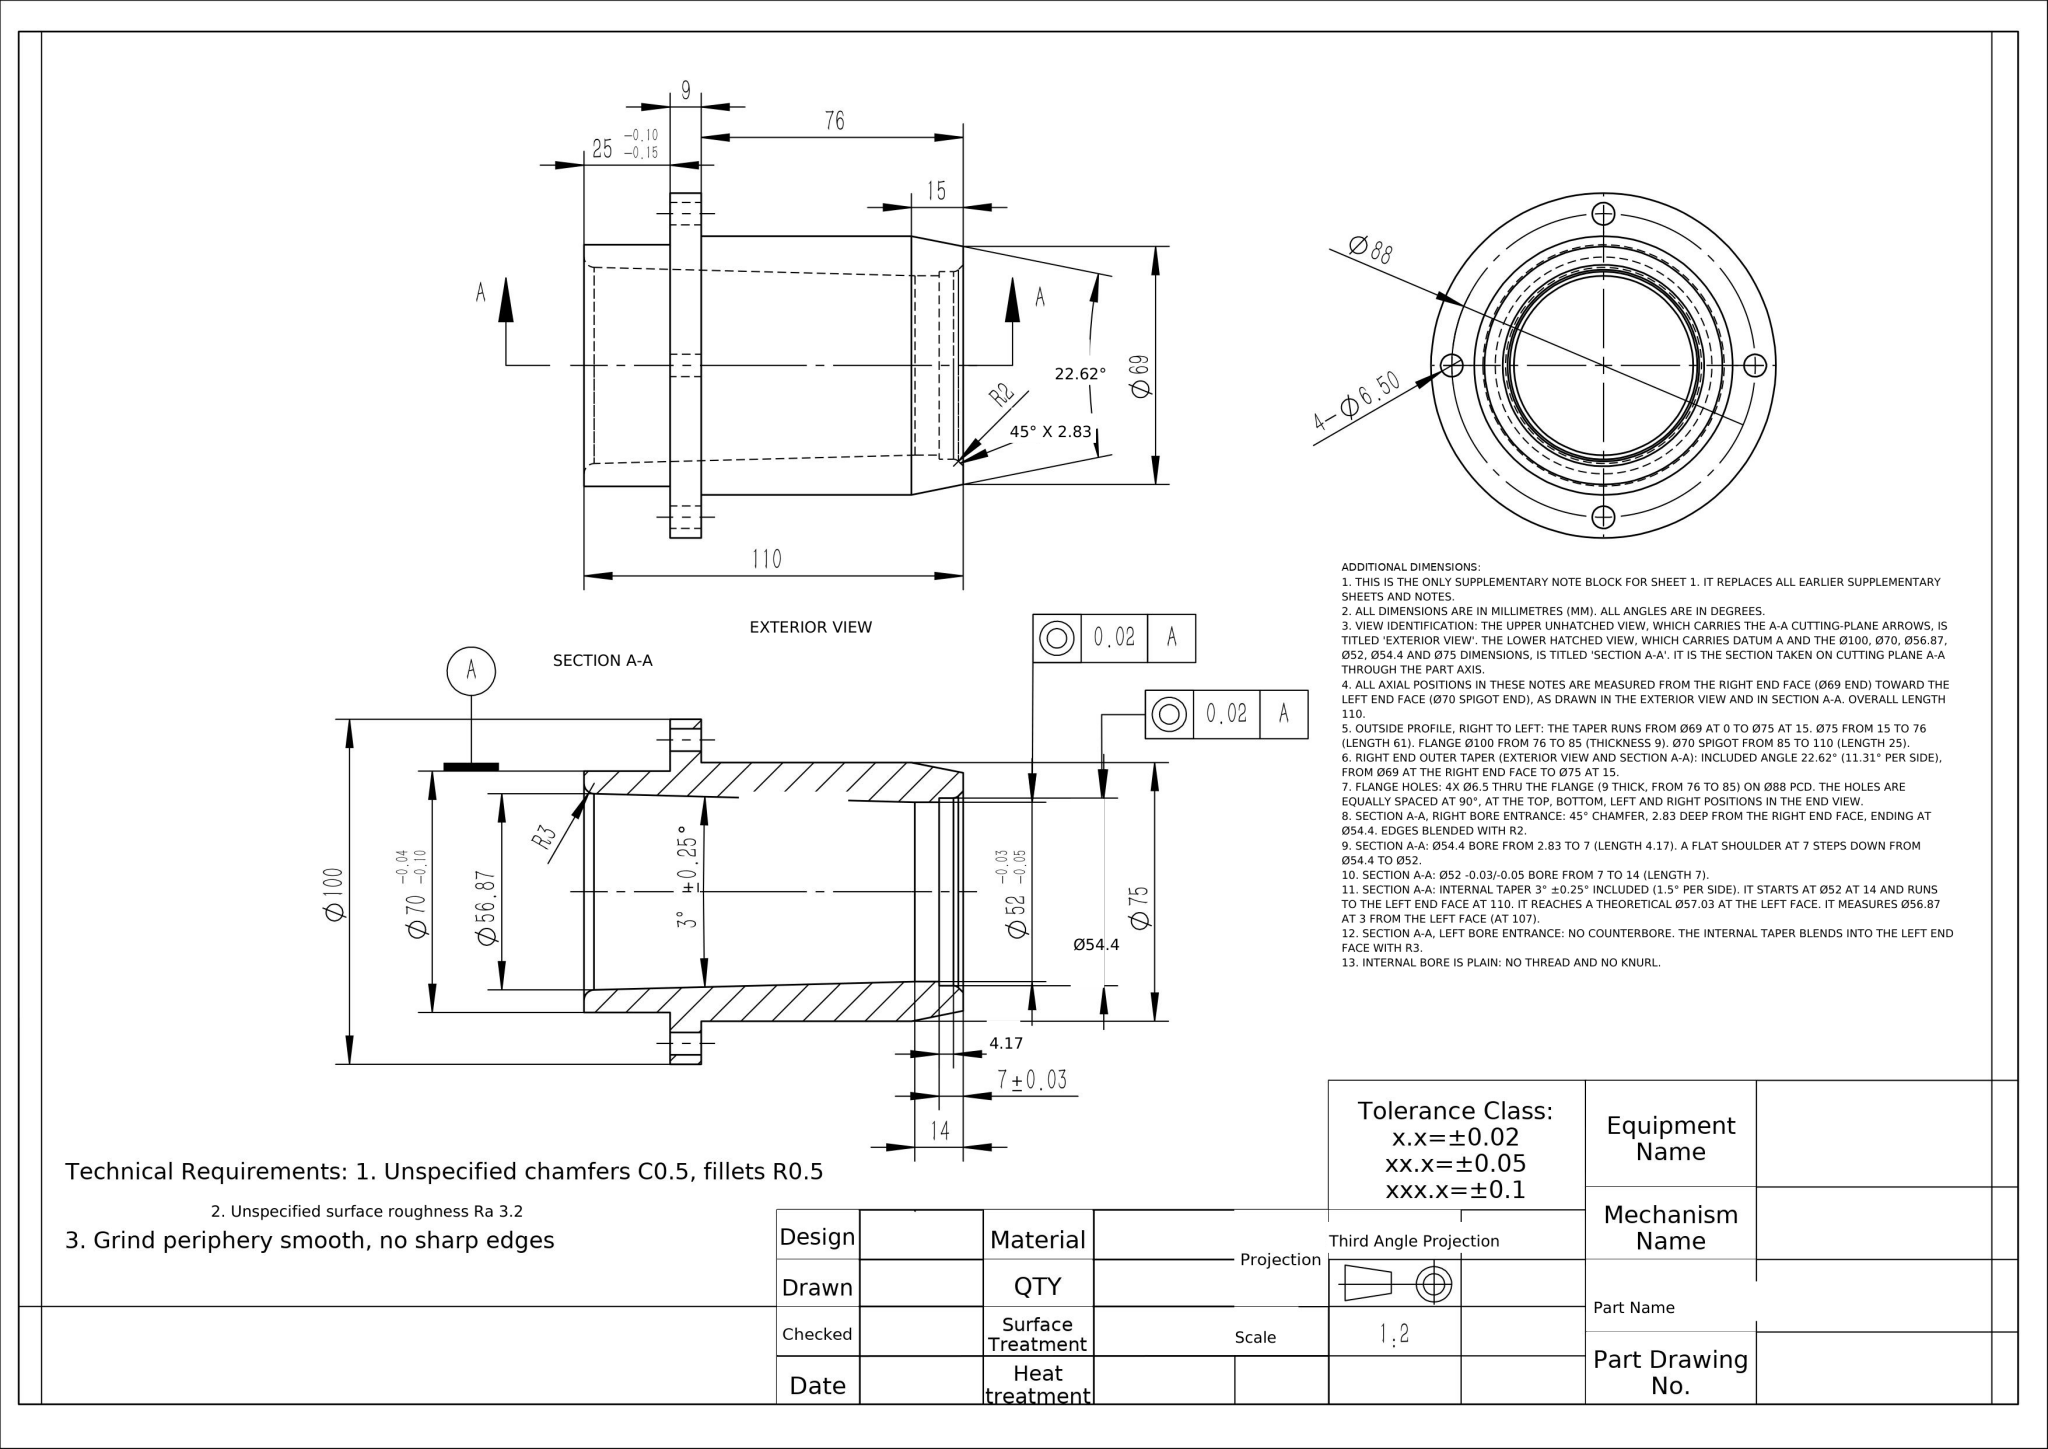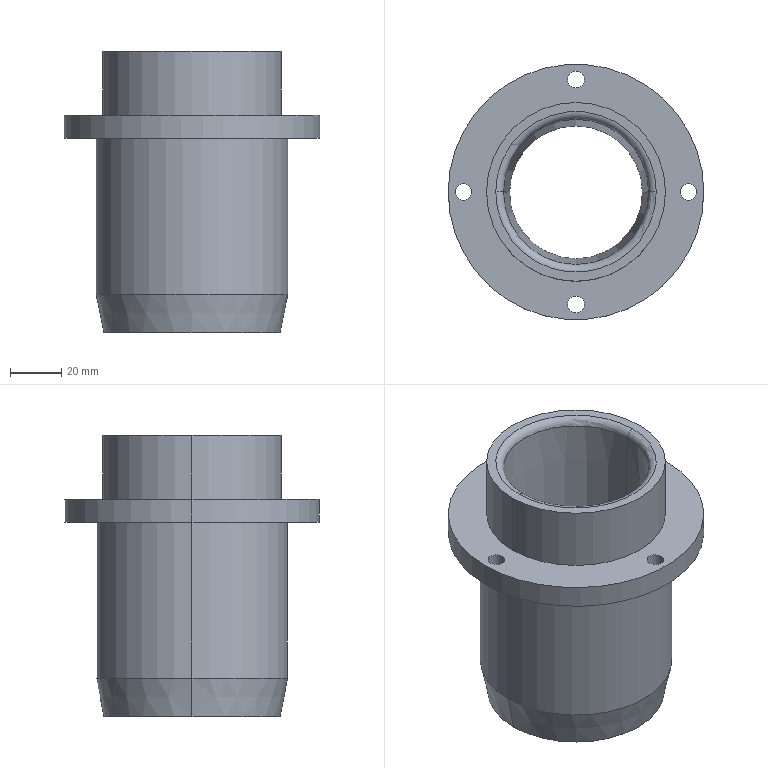Part | NX | mm | 1 solid | 33 faces | box 100 x 100 x 110 mm | volume 240242 mm3 | cylinder 18 | cone 6 | plane 5 | torus 4 | commonest cylinder face diameters 6.5 x8 54.4 x2 70 x2 100 x2 75 x2 52 x2
STEP:
#1=CARTESIAN_POINT('',(-27.2,0.,2.828));
#2=VERTEX_POINT('',#1);
#3=CARTESIAN_POINT('',(27.2,0.,2.828));
#4=VERTEX_POINT('',#3);
#5=CARTESIAN_POINT('',(0.,0.,2.828));
#6=DIRECTION('',(0.,0.,-1.));
#7=DIRECTION('',(1.,0.,0.));
#8=AXIS2_PLACEMENT_3D('',#5,#6,#7);
#9=CIRCLE('',#8,27.2);
#10=EDGE_CURVE('',#2,#4,#9,.T.);
#11=ORIENTED_EDGE('',*,*,#10,.F.);
#12=CARTESIAN_POINT('',(-27.786,0.,1.414));
#13=VERTEX_POINT('',#12);
#14=CARTESIAN_POINT('',(-29.2,0.,2.828));
#15=DIRECTION('',(0.,1.,0.));
#16=DIRECTION('',(-1.,0.,0.));
#17=AXIS2_PLACEMENT_3D('',#14,#15,#16);
#18=CIRCLE('',#17,2.);
#19=EDGE_CURVE('',#2,#13,#18,.T.);
#20=ORIENTED_EDGE('',*,*,#19,.T.);
#21=CARTESIAN_POINT('',(27.786,0.,1.414));
#22=VERTEX_POINT('',#21);
#23=CARTESIAN_POINT('',(0.,0.,1.414));
#24=DIRECTION('',(0.,0.,1.));
#25=DIRECTION('',(-1.,0.,0.));
#26=AXIS2_PLACEMENT_3D('',#23,#24,#25);
#27=CIRCLE('',#26,27.786);
#28=EDGE_CURVE('',#22,#13,#27,.T.);
#29=ORIENTED_EDGE('',*,*,#28,.F.);
#30=CARTESIAN_POINT('',(29.2,0.,2.828));
#31=DIRECTION('',(0.,-1.,0.));
#32=DIRECTION('',(0.,0.,-1.));
#33=AXIS2_PLACEMENT_3D('',#30,#31,#32);
#34=CIRCLE('',#33,2.);
#35=EDGE_CURVE('',#4,#22,#34,.T.);
#36=ORIENTED_EDGE('',*,*,#35,.F.);
#37=EDGE_LOOP('',(#11,#20,#29,#36));
#38=FACE_OUTER_BOUND('',#37,.T.);
#39=CARTESIAN_POINT('',(0.,0.,2.828));
#40=DIRECTION('',(0.,0.,1.));
#41=DIRECTION('',(1.,0.,0.));
#42=AXIS2_PLACEMENT_3D('',#39,#40,#41);
#43=TOROIDAL_SURFACE('',#42,29.2,2.);
#44=ADVANCED_FACE('',(#38),#43,.T.);
#45=CARTESIAN_POINT('',(-34.5,0.,0.));
#46=VERTEX_POINT('',#45);
#47=CARTESIAN_POINT('',(34.5,0.,0.));
#48=VERTEX_POINT('',#47);
#49=CARTESIAN_POINT('',(0.,0.,0.));
#50=DIRECTION('',(0.,0.,-1.));
#51=DIRECTION('',(1.,0.,0.));
#52=AXIS2_PLACEMENT_3D('',#49,#50,#51);
#53=CIRCLE('',#52,34.5);
#54=EDGE_CURVE('',#46,#48,#53,.T.);
#55=ORIENTED_EDGE('',*,*,#54,.F.);
#56=CARTESIAN_POINT('',(-37.5,0.,15.));
#57=VERTEX_POINT('',#56);
#58=CARTESIAN_POINT('',(-37.5,0.,15.));
#59=DIRECTION('',(-0.1961,0.,0.9806));
#60=VECTOR('',#59,1000.);
#61=LINE('',#58,#60);
#62=EDGE_CURVE('',#46,#57,#61,.T.);
#63=ORIENTED_EDGE('',*,*,#62,.T.);
#64=CARTESIAN_POINT('',(37.5,0.,15.));
#65=VERTEX_POINT('',#64);
#66=CARTESIAN_POINT('',(0.,0.,15.));
#67=DIRECTION('',(0.,0.,1.));
#68=DIRECTION('',(1.,0.,0.));
#69=AXIS2_PLACEMENT_3D('',#66,#67,#68);
#70=CIRCLE('',#69,37.5);
#71=EDGE_CURVE('',#65,#57,#70,.T.);
#72=ORIENTED_EDGE('',*,*,#71,.F.);
#73=CARTESIAN_POINT('',(37.5,0.,15.));
#74=DIRECTION('',(0.1961,0.,0.9806));
#75=VECTOR('',#74,1000.);
#76=LINE('',#73,#75);
#77=EDGE_CURVE('',#48,#65,#76,.T.);
#78=ORIENTED_EDGE('',*,*,#77,.F.);
#79=EDGE_LOOP('',(#55,#63,#72,#78));
#80=FACE_OUTER_BOUND('',#79,.T.);
#81=CARTESIAN_POINT('',(0.,0.,15.));
#82=DIRECTION('',(0.,0.,1.));
#83=DIRECTION('',(1.,0.,0.));
#84=AXIS2_PLACEMENT_3D('',#81,#82,#83);
#85=CONICAL_SURFACE('',#84,37.5,0.1974);
#86=ADVANCED_FACE('',(#80),#85,.T.);
#87=CARTESIAN_POINT('',(0.,0.,1.414));
#88=DIRECTION('',(0.,0.,1.));
#89=DIRECTION('',(-1.,0.,0.));
#90=AXIS2_PLACEMENT_3D('',#87,#88,#89);
#91=CIRCLE('',#90,27.786);
#92=EDGE_CURVE('',#13,#22,#91,.T.);
#93=ORIENTED_EDGE('',*,*,#92,.T.);
#94=CARTESIAN_POINT('',(29.2,0.,0.));
#95=VERTEX_POINT('',#94);
#96=CARTESIAN_POINT('',(27.2,0.,2.));
#97=DIRECTION('',(0.7071,0.,-0.7071));
#98=VECTOR('',#97,1000.);
#99=LINE('',#96,#98);
#100=EDGE_CURVE('',#22,#95,#99,.T.);
#101=ORIENTED_EDGE('',*,*,#100,.T.);
#102=CARTESIAN_POINT('',(-29.2,0.,0.));
#103=VERTEX_POINT('',#102);
#104=CARTESIAN_POINT('',(0.,0.,0.));
#105=DIRECTION('',(0.,0.,1.));
#106=DIRECTION('',(1.,0.,0.));
#107=AXIS2_PLACEMENT_3D('',#104,#105,#106);
#108=CIRCLE('',#107,29.2);
#109=EDGE_CURVE('',#103,#95,#108,.T.);
#110=ORIENTED_EDGE('',*,*,#109,.F.);
#111=CARTESIAN_POINT('',(-27.2,0.,2.));
#112=DIRECTION('',(-0.7071,0.,-0.7071));
#113=VECTOR('',#112,1000.);
#114=LINE('',#111,#113);
#115=EDGE_CURVE('',#13,#103,#114,.T.);
#116=ORIENTED_EDGE('',*,*,#115,.F.);
#117=EDGE_LOOP('',(#93,#101,#110,#116));
#118=FACE_OUTER_BOUND('',#117,.T.);
#119=CARTESIAN_POINT('',(0.,0.,2.));
#120=DIRECTION('',(0.,0.,-1.));
#121=DIRECTION('',(-1.,0.,0.));
#122=AXIS2_PLACEMENT_3D('',#119,#120,#121);
#123=CONICAL_SURFACE('',#122,27.2,0.7854);
#124=ADVANCED_FACE('',(#118),#123,.F.);
#125=CARTESIAN_POINT('',(-31.436,0.,110.));
#126=VERTEX_POINT('',#125);
#127=CARTESIAN_POINT('',(31.436,0.,110.));
#128=VERTEX_POINT('',#127);
#129=CARTESIAN_POINT('',(0.,0.,110.));
#130=DIRECTION('',(0.,0.,-1.));
#131=DIRECTION('',(1.,0.,0.));
#132=AXIS2_PLACEMENT_3D('',#129,#130,#131);
#133=CIRCLE('',#132,31.436);
#134=EDGE_CURVE('',#126,#128,#133,.T.);
#135=ORIENTED_EDGE('',*,*,#134,.F.);
#136=CARTESIAN_POINT('',(-28.437,0.,107.079));
#137=VERTEX_POINT('',#136);
#138=CARTESIAN_POINT('',(-31.436,0.,107.));
#139=DIRECTION('',(0.,1.,0.));
#140=DIRECTION('',(-1.,0.,0.));
#141=AXIS2_PLACEMENT_3D('',#138,#139,#140);
#142=CIRCLE('',#141,3.);
#143=EDGE_CURVE('',#126,#137,#142,.T.);
#144=ORIENTED_EDGE('',*,*,#143,.T.);
#145=CARTESIAN_POINT('',(28.437,0.,107.079));
#146=VERTEX_POINT('',#145);
#147=CARTESIAN_POINT('',(0.,0.,107.079));
#148=DIRECTION('',(0.,0.,1.));
#149=DIRECTION('',(-1.,0.,0.));
#150=AXIS2_PLACEMENT_3D('',#147,#148,#149);
#151=CIRCLE('',#150,28.437);
#152=EDGE_CURVE('',#146,#137,#151,.T.);
#153=ORIENTED_EDGE('',*,*,#152,.F.);
#154=CARTESIAN_POINT('',(31.436,0.,107.));
#155=DIRECTION('',(0.,-1.,0.));
#156=DIRECTION('',(0.,0.,-1.));
#157=AXIS2_PLACEMENT_3D('',#154,#155,#156);
#158=CIRCLE('',#157,3.);
#159=EDGE_CURVE('',#128,#146,#158,.T.);
#160=ORIENTED_EDGE('',*,*,#159,.F.);
#161=EDGE_LOOP('',(#135,#144,#153,#160));
#162=FACE_OUTER_BOUND('',#161,.T.);
#163=CARTESIAN_POINT('',(0.,0.,107.));
#164=DIRECTION('',(0.,0.,1.));
#165=DIRECTION('',(1.,0.,0.));
#166=AXIS2_PLACEMENT_3D('',#163,#164,#165);
#167=TOROIDAL_SURFACE('',#166,31.436,3.);
#168=ADVANCED_FACE('',(#162),#167,.T.);
#169=CARTESIAN_POINT('',(26.,0.,14.));
#170=VERTEX_POINT('',#169);
#171=CARTESIAN_POINT('',(-26.,0.,14.));
#172=VERTEX_POINT('',#171);
#173=CARTESIAN_POINT('',(0.,0.,14.));
#174=DIRECTION('',(0.,0.,-1.));
#175=DIRECTION('',(-1.,0.,0.));
#176=AXIS2_PLACEMENT_3D('',#173,#174,#175);
#177=CIRCLE('',#176,26.);
#178=EDGE_CURVE('',#170,#172,#177,.T.);
#179=ORIENTED_EDGE('',*,*,#178,.T.);
#180=CARTESIAN_POINT('',(-28.514,0.,110.));
#181=DIRECTION('',(-0.02618,0.,0.9997));
#182=VECTOR('',#181,1000.);
#183=LINE('',#180,#182);
#184=EDGE_CURVE('',#172,#137,#183,.T.);
#185=ORIENTED_EDGE('',*,*,#184,.T.);
#186=CARTESIAN_POINT('',(0.,0.,107.079));
#187=DIRECTION('',(0.,0.,1.));
#188=DIRECTION('',(-1.,0.,0.));
#189=AXIS2_PLACEMENT_3D('',#186,#187,#188);
#190=CIRCLE('',#189,28.437);
#191=EDGE_CURVE('',#137,#146,#190,.T.);
#192=ORIENTED_EDGE('',*,*,#191,.T.);
#193=CARTESIAN_POINT('',(28.514,0.,110.));
#194=DIRECTION('',(0.02618,0.,0.9997));
#195=VECTOR('',#194,1000.);
#196=LINE('',#193,#195);
#197=EDGE_CURVE('',#170,#146,#196,.T.);
#198=ORIENTED_EDGE('',*,*,#197,.F.);
#199=EDGE_LOOP('',(#179,#185,#192,#198));
#200=FACE_OUTER_BOUND('',#199,.T.);
#201=CARTESIAN_POINT('',(0.,0.,110.));
#202=DIRECTION('',(0.,0.,1.));
#203=DIRECTION('',(1.,0.,0.));
#204=AXIS2_PLACEMENT_3D('',#201,#202,#203);
#205=CONICAL_SURFACE('',#204,28.514,0.02618);
#206=ADVANCED_FACE('',(#200),#205,.F.);
#207=CARTESIAN_POINT('',(-3.25,44.,76.));
#208=VERTEX_POINT('',#207);
#209=CARTESIAN_POINT('',(3.25,44.,76.));
#210=VERTEX_POINT('',#209);
#211=CARTESIAN_POINT('',(0.,44.,76.));
#212=DIRECTION('',(0.,0.,1.));
#213=DIRECTION('',(1.,0.,0.));
#214=AXIS2_PLACEMENT_3D('',#211,#212,#213);
#215=CIRCLE('',#214,3.25);
#216=EDGE_CURVE('',#208,#210,#215,.T.);
#217=ORIENTED_EDGE('',*,*,#216,.F.);
#218=CARTESIAN_POINT('',(-3.25,44.,85.));
#219=VERTEX_POINT('',#218);
#220=CARTESIAN_POINT('',(-3.25,44.,85.));
#221=DIRECTION('',(0.,0.,1.));
#222=VECTOR('',#221,1000.);
#223=LINE('',#220,#222);
#224=EDGE_CURVE('',#208,#219,#223,.T.);
#225=ORIENTED_EDGE('',*,*,#224,.T.);
#226=CARTESIAN_POINT('',(3.25,44.,85.));
#227=VERTEX_POINT('',#226);
#228=CARTESIAN_POINT('',(0.,44.,85.));
#229=DIRECTION('',(0.,0.,1.));
#230=DIRECTION('',(1.,0.,0.));
#231=AXIS2_PLACEMENT_3D('',#228,#229,#230);
#232=CIRCLE('',#231,3.25);
#233=EDGE_CURVE('',#219,#227,#232,.T.);
#234=ORIENTED_EDGE('',*,*,#233,.T.);
#235=CARTESIAN_POINT('',(3.25,44.,85.));
#236=DIRECTION('',(0.,0.,1.));
#237=VECTOR('',#236,1000.);
#238=LINE('',#235,#237);
#239=EDGE_CURVE('',#210,#227,#238,.T.);
#240=ORIENTED_EDGE('',*,*,#239,.F.);
#241=EDGE_LOOP('',(#217,#225,#234,#240));
#242=FACE_OUTER_BOUND('',#241,.T.);
#243=CARTESIAN_POINT('',(0.,44.,85.));
#244=DIRECTION('',(0.,0.,1.));
#245=DIRECTION('',(1.,0.,0.));
#246=AXIS2_PLACEMENT_3D('',#243,#244,#245);
#247=CYLINDRICAL_SURFACE('',#246,3.25);
#248=ADVANCED_FACE('',(#242),#247,.F.);
#249=CARTESIAN_POINT('',(-47.25,0.,76.));
#250=VERTEX_POINT('',#249);
#251=CARTESIAN_POINT('',(-40.75,0.,76.));
#252=VERTEX_POINT('',#251);
#253=CARTESIAN_POINT('',(-44.,0.,76.));
#254=DIRECTION('',(0.,0.,1.));
#255=DIRECTION('',(1.,0.,0.));
#256=AXIS2_PLACEMENT_3D('',#253,#254,#255);
#257=CIRCLE('',#256,3.25);
#258=EDGE_CURVE('',#250,#252,#257,.T.);
#259=ORIENTED_EDGE('',*,*,#258,.F.);
#260=CARTESIAN_POINT('',(-47.25,0.,85.));
#261=VERTEX_POINT('',#260);
#262=CARTESIAN_POINT('',(-47.25,0.,85.));
#263=DIRECTION('',(0.,0.,1.));
#264=VECTOR('',#263,1000.);
#265=LINE('',#262,#264);
#266=EDGE_CURVE('',#250,#261,#265,.T.);
#267=ORIENTED_EDGE('',*,*,#266,.T.);
#268=CARTESIAN_POINT('',(-40.75,0.,85.));
#269=VERTEX_POINT('',#268);
#270=CARTESIAN_POINT('',(-44.,0.,85.));
#271=DIRECTION('',(0.,0.,1.));
#272=DIRECTION('',(1.,0.,0.));
#273=AXIS2_PLACEMENT_3D('',#270,#271,#272);
#274=CIRCLE('',#273,3.25);
#275=EDGE_CURVE('',#261,#269,#274,.T.);
#276=ORIENTED_EDGE('',*,*,#275,.T.);
#277=CARTESIAN_POINT('',(-40.75,0.,85.));
#278=DIRECTION('',(0.,0.,1.));
#279=VECTOR('',#278,1000.);
#280=LINE('',#277,#279);
#281=EDGE_CURVE('',#252,#269,#280,.T.);
#282=ORIENTED_EDGE('',*,*,#281,.F.);
#283=EDGE_LOOP('',(#259,#267,#276,#282));
#284=FACE_OUTER_BOUND('',#283,.T.);
#285=CARTESIAN_POINT('',(-44.,0.,85.));
#286=DIRECTION('',(0.,0.,1.));
#287=DIRECTION('',(1.,0.,0.));
#288=AXIS2_PLACEMENT_3D('',#285,#286,#287);
#289=CYLINDRICAL_SURFACE('',#288,3.25);
#290=ADVANCED_FACE('',(#284),#289,.F.);
#291=CARTESIAN_POINT('',(-3.25,-44.,76.));
#292=VERTEX_POINT('',#291);
#293=CARTESIAN_POINT('',(3.25,-44.,76.));
#294=VERTEX_POINT('',#293);
#295=CARTESIAN_POINT('',(-0.,-44.,76.));
#296=DIRECTION('',(0.,0.,1.));
#297=DIRECTION('',(1.,0.,0.));
#298=AXIS2_PLACEMENT_3D('',#295,#296,#297);
#299=CIRCLE('',#298,3.25);
#300=EDGE_CURVE('',#292,#294,#299,.T.);
#301=ORIENTED_EDGE('',*,*,#300,.F.);
#302=CARTESIAN_POINT('',(-3.25,-44.,85.));
#303=VERTEX_POINT('',#302);
#304=CARTESIAN_POINT('',(-3.25,-44.,85.));
#305=DIRECTION('',(0.,0.,1.));
#306=VECTOR('',#305,1000.);
#307=LINE('',#304,#306);
#308=EDGE_CURVE('',#292,#303,#307,.T.);
#309=ORIENTED_EDGE('',*,*,#308,.T.);
#310=CARTESIAN_POINT('',(3.25,-44.,85.));
#311=VERTEX_POINT('',#310);
#312=CARTESIAN_POINT('',(-0.,-44.,85.));
#313=DIRECTION('',(0.,0.,1.));
#314=DIRECTION('',(1.,0.,0.));
#315=AXIS2_PLACEMENT_3D('',#312,#313,#314);
#316=CIRCLE('',#315,3.25);
#317=EDGE_CURVE('',#303,#311,#316,.T.);
#318=ORIENTED_EDGE('',*,*,#317,.T.);
#319=CARTESIAN_POINT('',(3.25,-44.,85.));
#320=DIRECTION('',(0.,0.,1.));
#321=VECTOR('',#320,1000.);
#322=LINE('',#319,#321);
#323=EDGE_CURVE('',#294,#311,#322,.T.);
#324=ORIENTED_EDGE('',*,*,#323,.F.);
#325=EDGE_LOOP('',(#301,#309,#318,#324));
#326=FACE_OUTER_BOUND('',#325,.T.);
#327=CARTESIAN_POINT('',(-0.,-44.,85.));
#328=DIRECTION('',(0.,0.,1.));
#329=DIRECTION('',(1.,0.,0.));
#330=AXIS2_PLACEMENT_3D('',#327,#328,#329);
#331=CYLINDRICAL_SURFACE('',#330,3.25);
#332=ADVANCED_FACE('',(#326),#331,.F.);
#333=CARTESIAN_POINT('',(40.75,0.,76.));
#334=VERTEX_POINT('',#333);
#335=CARTESIAN_POINT('',(47.25,0.,76.));
#336=VERTEX_POINT('',#335);
#337=CARTESIAN_POINT('',(44.,0.,76.));
#338=DIRECTION('',(0.,0.,1.));
#339=DIRECTION('',(1.,0.,0.));
#340=AXIS2_PLACEMENT_3D('',#337,#338,#339);
#341=CIRCLE('',#340,3.25);
#342=EDGE_CURVE('',#334,#336,#341,.T.);
#343=ORIENTED_EDGE('',*,*,#342,.F.);
#344=CARTESIAN_POINT('',(40.75,0.,85.));
#345=VERTEX_POINT('',#344);
#346=CARTESIAN_POINT('',(40.75,0.,85.));
#347=DIRECTION('',(0.,0.,1.));
#348=VECTOR('',#347,1000.);
#349=LINE('',#346,#348);
#350=EDGE_CURVE('',#334,#345,#349,.T.);
#351=ORIENTED_EDGE('',*,*,#350,.T.);
#352=CARTESIAN_POINT('',(47.25,0.,85.));
#353=VERTEX_POINT('',#352);
#354=CARTESIAN_POINT('',(44.,0.,85.));
#355=DIRECTION('',(0.,0.,1.));
#356=DIRECTION('',(1.,0.,0.));
#357=AXIS2_PLACEMENT_3D('',#354,#355,#356);
#358=CIRCLE('',#357,3.25);
#359=EDGE_CURVE('',#345,#353,#358,.T.);
#360=ORIENTED_EDGE('',*,*,#359,.T.);
#361=CARTESIAN_POINT('',(47.25,0.,85.));
#362=DIRECTION('',(0.,0.,1.));
#363=VECTOR('',#362,1000.);
#364=LINE('',#361,#363);
#365=EDGE_CURVE('',#336,#353,#364,.T.);
#366=ORIENTED_EDGE('',*,*,#365,.F.);
#367=EDGE_LOOP('',(#343,#351,#360,#366));
#368=FACE_OUTER_BOUND('',#367,.T.);
#369=CARTESIAN_POINT('',(44.,0.,85.));
#370=DIRECTION('',(0.,0.,1.));
#371=DIRECTION('',(1.,0.,0.));
#372=AXIS2_PLACEMENT_3D('',#369,#370,#371);
#373=CYLINDRICAL_SURFACE('',#372,3.25);
#374=ADVANCED_FACE('',(#368),#373,.F.);
#375=CARTESIAN_POINT('',(27.2,0.,7.));
#376=VERTEX_POINT('',#375);
#377=CARTESIAN_POINT('',(-27.2,0.,7.));
#378=VERTEX_POINT('',#377);
#379=CARTESIAN_POINT('',(0.,0.,7.));
#380=DIRECTION('',(0.,0.,-1.));
#381=DIRECTION('',(-1.,0.,0.));
#382=AXIS2_PLACEMENT_3D('',#379,#380,#381);
#383=CIRCLE('',#382,27.2);
#384=EDGE_CURVE('',#376,#378,#383,.T.);
#385=ORIENTED_EDGE('',*,*,#384,.F.);
#386=CARTESIAN_POINT('',(27.2,0.,7.));
#387=DIRECTION('',(0.,0.,-1.));
#388=VECTOR('',#387,1000.);
#389=LINE('',#386,#388);
#390=EDGE_CURVE('',#376,#4,#389,.T.);
#391=ORIENTED_EDGE('',*,*,#390,.T.);
#392=CARTESIAN_POINT('',(0.,0.,2.828));
#393=DIRECTION('',(0.,0.,-1.));
#394=DIRECTION('',(1.,0.,0.));
#395=AXIS2_PLACEMENT_3D('',#392,#393,#394);
#396=CIRCLE('',#395,27.2);
#397=EDGE_CURVE('',#4,#2,#396,.T.);
#398=ORIENTED_EDGE('',*,*,#397,.T.);
#399=CARTESIAN_POINT('',(-27.2,0.,7.));
#400=DIRECTION('',(0.,0.,-1.));
#401=VECTOR('',#400,1000.);
#402=LINE('',#399,#401);
#403=EDGE_CURVE('',#378,#2,#402,.T.);
#404=ORIENTED_EDGE('',*,*,#403,.F.);
#405=EDGE_LOOP('',(#385,#391,#398,#404));
#406=FACE_OUTER_BOUND('',#405,.T.);
#407=CARTESIAN_POINT('',(0.,0.,7.));
#408=DIRECTION('',(0.,0.,-1.));
#409=DIRECTION('',(-1.,0.,0.));
#410=AXIS2_PLACEMENT_3D('',#407,#408,#409);
#411=CYLINDRICAL_SURFACE('',#410,27.2);
#412=ADVANCED_FACE('',(#406),#411,.F.);
#413=CARTESIAN_POINT('',(35.,0.,110.));
#414=VERTEX_POINT('',#413);
#415=CARTESIAN_POINT('',(-35.,0.,110.));
#416=VERTEX_POINT('',#415);
#417=CARTESIAN_POINT('',(0.,0.,110.));
#418=DIRECTION('',(0.,0.,1.));
#419=DIRECTION('',(1.,0.,0.));
#420=AXIS2_PLACEMENT_3D('',#417,#418,#419);
#421=CIRCLE('',#420,35.);
#422=EDGE_CURVE('',#414,#416,#421,.T.);
#423=ORIENTED_EDGE('',*,*,#422,.F.);
#424=CARTESIAN_POINT('',(35.,0.,85.));
#425=VERTEX_POINT('',#424);
#426=CARTESIAN_POINT('',(35.,0.,110.));
#427=DIRECTION('',(0.,0.,-1.));
#428=VECTOR('',#427,1000.);
#429=LINE('',#426,#428);
#430=EDGE_CURVE('',#414,#425,#429,.T.);
#431=ORIENTED_EDGE('',*,*,#430,.T.);
#432=CARTESIAN_POINT('',(-35.,0.,85.));
#433=VERTEX_POINT('',#432);
#434=CARTESIAN_POINT('',(0.,0.,85.));
#435=DIRECTION('',(0.,0.,1.));
#436=DIRECTION('',(1.,0.,0.));
#437=AXIS2_PLACEMENT_3D('',#434,#435,#436);
#438=CIRCLE('',#437,35.);
#439=EDGE_CURVE('',#425,#433,#438,.T.);
#440=ORIENTED_EDGE('',*,*,#439,.T.);
#441=CARTESIAN_POINT('',(-35.,0.,110.));
#442=DIRECTION('',(0.,0.,-1.));
#443=VECTOR('',#442,1000.);
#444=LINE('',#441,#443);
#445=EDGE_CURVE('',#416,#433,#444,.T.);
#446=ORIENTED_EDGE('',*,*,#445,.F.);
#447=EDGE_LOOP('',(#423,#431,#440,#446));
#448=FACE_OUTER_BOUND('',#447,.T.);
#449=CARTESIAN_POINT('',(0.,0.,110.));
#450=DIRECTION('',(0.,0.,-1.));
#451=DIRECTION('',(-1.,0.,0.));
#452=AXIS2_PLACEMENT_3D('',#449,#450,#451);
#453=CYLINDRICAL_SURFACE('',#452,35.);
#454=ADVANCED_FACE('',(#448),#453,.T.);
#455=CARTESIAN_POINT('',(50.,0.,85.));
#456=VERTEX_POINT('',#455);
#457=CARTESIAN_POINT('',(-50.,0.,85.));
#458=VERTEX_POINT('',#457);
#459=CARTESIAN_POINT('',(0.,0.,85.));
#460=DIRECTION('',(0.,0.,1.));
#461=DIRECTION('',(1.,0.,0.));
#462=AXIS2_PLACEMENT_3D('',#459,#460,#461);
#463=CIRCLE('',#462,50.);
#464=EDGE_CURVE('',#456,#458,#463,.T.);
#465=ORIENTED_EDGE('',*,*,#464,.F.);
#466=CARTESIAN_POINT('',(50.,0.,76.));
#467=VERTEX_POINT('',#466);
#468=CARTESIAN_POINT('',(50.,0.,85.));
#469=DIRECTION('',(0.,0.,-1.));
#470=VECTOR('',#469,1000.);
#471=LINE('',#468,#470);
#472=EDGE_CURVE('',#456,#467,#471,.T.);
#473=ORIENTED_EDGE('',*,*,#472,.T.);
#474=CARTESIAN_POINT('',(-50.,0.,76.));
#475=VERTEX_POINT('',#474);
#476=CARTESIAN_POINT('',(0.,0.,76.));
#477=DIRECTION('',(0.,0.,1.));
#478=DIRECTION('',(1.,0.,0.));
#479=AXIS2_PLACEMENT_3D('',#476,#477,#478);
#480=CIRCLE('',#479,50.);
#481=EDGE_CURVE('',#467,#475,#480,.T.);
#482=ORIENTED_EDGE('',*,*,#481,.T.);
#483=CARTESIAN_POINT('',(-50.,0.,85.));
#484=DIRECTION('',(0.,0.,-1.));
#485=VECTOR('',#484,1000.);
#486=LINE('',#483,#485);
#487=EDGE_CURVE('',#458,#475,#486,.T.);
#488=ORIENTED_EDGE('',*,*,#487,.F.);
#489=EDGE_LOOP('',(#465,#473,#482,#488));
#490=FACE_OUTER_BOUND('',#489,.T.);
#491=CARTESIAN_POINT('',(0.,0.,85.));
#492=DIRECTION('',(0.,0.,-1.));
#493=DIRECTION('',(-1.,0.,0.));
#494=AXIS2_PLACEMENT_3D('',#491,#492,#493);
#495=CYLINDRICAL_SURFACE('',#494,50.);
#496=ADVANCED_FACE('',(#490),#495,.T.);
#497=CARTESIAN_POINT('',(37.5,0.,76.));
#498=VERTEX_POINT('',#497);
#499=CARTESIAN_POINT('',(-37.5,0.,76.));
#500=VERTEX_POINT('',#499);
#501=CARTESIAN_POINT('',(0.,0.,76.));
#502=DIRECTION('',(0.,0.,1.));
#503=DIRECTION('',(1.,0.,0.));
#504=AXIS2_PLACEMENT_3D('',#501,#502,#503);
#505=CIRCLE('',#504,37.5);
#506=EDGE_CURVE('',#498,#500,#505,.T.);
#507=ORIENTED_EDGE('',*,*,#506,.F.);
#508=CARTESIAN_POINT('',(37.5,0.,76.));
#509=DIRECTION('',(0.,0.,-1.));
#510=VECTOR('',#509,1000.);
#511=LINE('',#508,#510);
#512=EDGE_CURVE('',#498,#65,#511,.T.);
#513=ORIENTED_EDGE('',*,*,#512,.T.);
#514=ORIENTED_EDGE('',*,*,#71,.T.);
#515=CARTESIAN_POINT('',(-37.5,0.,76.));
#516=DIRECTION('',(0.,0.,-1.));
#517=VECTOR('',#516,1000.);
#518=LINE('',#515,#517);
#519=EDGE_CURVE('',#500,#57,#518,.T.);
#520=ORIENTED_EDGE('',*,*,#519,.F.);
#521=EDGE_LOOP('',(#507,#513,#514,#520));
#522=FACE_OUTER_BOUND('',#521,.T.);
#523=CARTESIAN_POINT('',(0.,0.,76.));
#524=DIRECTION('',(0.,0.,-1.));
#525=DIRECTION('',(-1.,0.,0.));
#526=AXIS2_PLACEMENT_3D('',#523,#524,#525);
#527=CYLINDRICAL_SURFACE('',#526,37.5);
#528=ADVANCED_FACE('',(#522),#527,.T.);
#529=CARTESIAN_POINT('',(-26.,0.,7.));
#530=VERTEX_POINT('',#529);
#531=CARTESIAN_POINT('',(26.,0.,7.));
#532=VERTEX_POINT('',#531);
#533=CARTESIAN_POINT('',(0.,0.,7.));
#534=DIRECTION('',(0.,0.,1.));
#535=DIRECTION('',(-1.,0.,0.));
#536=AXIS2_PLACEMENT_3D('',#533,#534,#535);
#537=CIRCLE('',#536,26.);
#538=EDGE_CURVE('',#530,#532,#537,.T.);
#539=ORIENTED_EDGE('',*,*,#538,.F.);
#540=CARTESIAN_POINT('',(-26.,0.,0.));
#541=DIRECTION('',(0.,0.,1.));
#542=VECTOR('',#541,1000.);
#543=LINE('',#540,#542);
#544=EDGE_CURVE('',#530,#172,#543,.T.);
#545=ORIENTED_EDGE('',*,*,#544,.T.);
#546=ORIENTED_EDGE('',*,*,#178,.F.);
#547=CARTESIAN_POINT('',(26.,0.,0.));
#548=DIRECTION('',(0.,0.,1.));
#549=VECTOR('',#548,1000.);
#550=LINE('',#547,#549);
#551=EDGE_CURVE('',#532,#170,#550,.T.);
#552=ORIENTED_EDGE('',*,*,#551,.F.);
#553=EDGE_LOOP('',(#539,#545,#546,#552));
#554=FACE_OUTER_BOUND('',#553,.T.);
#555=CARTESIAN_POINT('',(0.,0.,0.));
#556=DIRECTION('',(0.,0.,1.));
#557=DIRECTION('',(1.,0.,0.));
#558=AXIS2_PLACEMENT_3D('',#555,#556,#557);
#559=CYLINDRICAL_SURFACE('',#558,26.);
#560=ADVANCED_FACE('',(#554),#559,.F.);
#561=ORIENTED_EDGE('',*,*,#544,.F.);
#562=CARTESIAN_POINT('',(0.,0.,7.));
#563=DIRECTION('',(0.,0.,1.));
#564=DIRECTION('',(-1.,0.,0.));
#565=AXIS2_PLACEMENT_3D('',#562,#563,#564);
#566=CIRCLE('',#565,26.);
#567=EDGE_CURVE('',#532,#530,#566,.T.);
#568=ORIENTED_EDGE('',*,*,#567,.F.);
#569=ORIENTED_EDGE('',*,*,#551,.T.);
#570=CARTESIAN_POINT('',(0.,0.,14.));
#571=DIRECTION('',(0.,0.,-1.));
#572=DIRECTION('',(-1.,0.,0.));
#573=AXIS2_PLACEMENT_3D('',#570,#571,#572);
#574=CIRCLE('',#573,26.);
#575=EDGE_CURVE('',#172,#170,#574,.T.);
#576=ORIENTED_EDGE('',*,*,#575,.F.);
#577=EDGE_LOOP('',(#561,#568,#569,#576));
#578=FACE_OUTER_BOUND('',#577,.T.);
#579=CARTESIAN_POINT('',(0.,0.,0.));
#580=DIRECTION('',(0.,0.,1.));
#581=DIRECTION('',(1.,0.,0.));
#582=AXIS2_PLACEMENT_3D('',#579,#580,#581);
#583=CYLINDRICAL_SURFACE('',#582,26.);
#584=ADVANCED_FACE('',(#578),#583,.F.);
#585=CARTESIAN_POINT('',(0.,0.,110.));
#586=DIRECTION('',(0.,0.,-1.));
#587=DIRECTION('',(1.,0.,0.));
#588=AXIS2_PLACEMENT_3D('',#585,#586,#587);
#589=CIRCLE('',#588,31.436);
#590=EDGE_CURVE('',#128,#126,#589,.T.);
#591=ORIENTED_EDGE('',*,*,#590,.T.);
#592=ORIENTED_EDGE('',*,*,#134,.T.);
#593=EDGE_LOOP('',(#591,#592));
#594=FACE_BOUND('',#593,.T.);
#595=CARTESIAN_POINT('',(0.,0.,110.));
#596=DIRECTION('',(0.,0.,1.));
#597=DIRECTION('',(1.,0.,0.));
#598=AXIS2_PLACEMENT_3D('',#595,#596,#597);
#599=CIRCLE('',#598,35.);
#600=EDGE_CURVE('',#416,#414,#599,.T.);
#601=ORIENTED_EDGE('',*,*,#600,.T.);
#602=ORIENTED_EDGE('',*,*,#422,.T.);
#603=EDGE_LOOP('',(#601,#602));
#604=FACE_OUTER_BOUND('',#603,.T.);
#605=CARTESIAN_POINT('',(0.,0.,110.));
#606=DIRECTION('',(0.,0.,1.));
#607=DIRECTION('',(1.,0.,0.));
#608=AXIS2_PLACEMENT_3D('',#605,#606,#607);
#609=PLANE('',#608);
#610=ADVANCED_FACE('',(#594,#604),#609,.T.);
#611=CARTESIAN_POINT('',(0.,44.,85.));
#612=DIRECTION('',(0.,0.,1.));
#613=DIRECTION('',(1.,0.,0.));
#614=AXIS2_PLACEMENT_3D('',#611,#612,#613);
#615=CIRCLE('',#614,3.25);
#616=EDGE_CURVE('',#227,#219,#615,.T.);
#617=ORIENTED_EDGE('',*,*,#616,.F.);
#618=ORIENTED_EDGE('',*,*,#233,.F.);
#619=EDGE_LOOP('',(#617,#618));
#620=FACE_BOUND('',#619,.T.);
#621=CARTESIAN_POINT('',(-44.,0.,85.));
#622=DIRECTION('',(0.,0.,1.));
#623=DIRECTION('',(1.,0.,0.));
#624=AXIS2_PLACEMENT_3D('',#621,#622,#623);
#625=CIRCLE('',#624,3.25);
#626=EDGE_CURVE('',#269,#261,#625,.T.);
#627=ORIENTED_EDGE('',*,*,#626,.F.);
#628=ORIENTED_EDGE('',*,*,#275,.F.);
#629=EDGE_LOOP('',(#627,#628));
#630=FACE_BOUND('',#629,.T.);
#631=CARTESIAN_POINT('',(-0.,-44.,85.));
#632=DIRECTION('',(0.,0.,1.));
#633=DIRECTION('',(1.,0.,0.));
#634=AXIS2_PLACEMENT_3D('',#631,#632,#633);
#635=CIRCLE('',#634,3.25);
#636=EDGE_CURVE('',#311,#303,#635,.T.);
#637=ORIENTED_EDGE('',*,*,#636,.F.);
#638=ORIENTED_EDGE('',*,*,#317,.F.);
#639=EDGE_LOOP('',(#637,#638));
#640=FACE_BOUND('',#639,.T.);
#641=CARTESIAN_POINT('',(44.,0.,85.));
#642=DIRECTION('',(0.,0.,1.));
#643=DIRECTION('',(1.,0.,0.));
#644=AXIS2_PLACEMENT_3D('',#641,#642,#643);
#645=CIRCLE('',#644,3.25);
#646=EDGE_CURVE('',#353,#345,#645,.T.);
#647=ORIENTED_EDGE('',*,*,#646,.F.);
#648=ORIENTED_EDGE('',*,*,#359,.F.);
#649=EDGE_LOOP('',(#647,#648));
#650=FACE_BOUND('',#649,.T.);
#651=CARTESIAN_POINT('',(0.,0.,85.));
#652=DIRECTION('',(0.,0.,1.));
#653=DIRECTION('',(1.,0.,0.));
#654=AXIS2_PLACEMENT_3D('',#651,#652,#653);
#655=CIRCLE('',#654,50.);
#656=EDGE_CURVE('',#458,#456,#655,.T.);
#657=ORIENTED_EDGE('',*,*,#656,.T.);
#658=ORIENTED_EDGE('',*,*,#464,.T.);
#659=EDGE_LOOP('',(#657,#658));
#660=FACE_OUTER_BOUND('',#659,.T.);
#661=CARTESIAN_POINT('',(0.,0.,85.));
#662=DIRECTION('',(0.,0.,1.));
#663=DIRECTION('',(1.,0.,0.));
#664=AXIS2_PLACEMENT_3D('',#661,#662,#663);
#665=CIRCLE('',#664,35.);
#666=EDGE_CURVE('',#433,#425,#665,.T.);
#667=ORIENTED_EDGE('',*,*,#666,.F.);
#668=ORIENTED_EDGE('',*,*,#439,.F.);
#669=EDGE_LOOP('',(#667,#668));
#670=FACE_BOUND('',#669,.T.);
#671=CARTESIAN_POINT('',(0.,0.,85.));
#672=DIRECTION('',(0.,0.,1.));
#673=DIRECTION('',(1.,0.,0.));
#674=AXIS2_PLACEMENT_3D('',#671,#672,#673);
#675=PLANE('',#674);
#676=ADVANCED_FACE('',(#620,#630,#640,#650,#660,#670),#675,.T.);
#677=ORIENTED_EDGE('',*,*,#512,.F.);
#678=CARTESIAN_POINT('',(0.,0.,76.));
#679=DIRECTION('',(0.,0.,1.));
#680=DIRECTION('',(1.,0.,0.));
#681=AXIS2_PLACEMENT_3D('',#678,#679,#680);
#682=CIRCLE('',#681,37.5);
#683=EDGE_CURVE('',#500,#498,#682,.T.);
#684=ORIENTED_EDGE('',*,*,#683,.F.);
#685=ORIENTED_EDGE('',*,*,#519,.T.);
#686=CARTESIAN_POINT('',(0.,0.,15.));
#687=DIRECTION('',(0.,0.,1.));
#688=DIRECTION('',(1.,0.,0.));
#689=AXIS2_PLACEMENT_3D('',#686,#687,#688);
#690=CIRCLE('',#689,37.5);
#691=EDGE_CURVE('',#57,#65,#690,.T.);
#692=ORIENTED_EDGE('',*,*,#691,.T.);
#693=EDGE_LOOP('',(#677,#684,#685,#692));
#694=FACE_OUTER_BOUND('',#693,.T.);
#695=CARTESIAN_POINT('',(0.,0.,76.));
#696=DIRECTION('',(0.,0.,-1.));
#697=DIRECTION('',(-1.,0.,0.));
#698=AXIS2_PLACEMENT_3D('',#695,#696,#697);
#699=CYLINDRICAL_SURFACE('',#698,37.5);
#700=ADVANCED_FACE('',(#694),#699,.T.);
#701=CARTESIAN_POINT('',(0.,0.,0.));
#702=DIRECTION('',(0.,0.,-1.));
#703=DIRECTION('',(1.,0.,0.));
#704=AXIS2_PLACEMENT_3D('',#701,#702,#703);
#705=CIRCLE('',#704,34.5);
#706=EDGE_CURVE('',#48,#46,#705,.T.);
#707=ORIENTED_EDGE('',*,*,#706,.T.);
#708=ORIENTED_EDGE('',*,*,#54,.T.);
#709=EDGE_LOOP('',(#707,#708));
#710=FACE_OUTER_BOUND('',#709,.T.);
#711=ORIENTED_EDGE('',*,*,#109,.T.);
#712=CARTESIAN_POINT('',(0.,0.,0.));
#713=DIRECTION('',(0.,0.,1.));
#714=DIRECTION('',(1.,0.,0.));
#715=AXIS2_PLACEMENT_3D('',#712,#713,#714);
#716=CIRCLE('',#715,29.2);
#717=EDGE_CURVE('',#95,#103,#716,.T.);
#718=ORIENTED_EDGE('',*,*,#717,.T.);
#719=EDGE_LOOP('',(#711,#718));
#720=FACE_BOUND('',#719,.T.);
#721=CARTESIAN_POINT('',(0.,0.,0.));
#722=DIRECTION('',(0.,0.,1.));
#723=DIRECTION('',(1.,0.,0.));
#724=AXIS2_PLACEMENT_3D('',#721,#722,#723);
#725=PLANE('',#724);
#726=ADVANCED_FACE('',(#710,#720),#725,.F.);
#727=CARTESIAN_POINT('',(0.,44.,76.));
#728=DIRECTION('',(0.,0.,1.));
#729=DIRECTION('',(1.,0.,0.));
#730=AXIS2_PLACEMENT_3D('',#727,#728,#729);
#731=CIRCLE('',#730,3.25);
#732=EDGE_CURVE('',#210,#208,#731,.T.);
#733=ORIENTED_EDGE('',*,*,#732,.T.);
#734=ORIENTED_EDGE('',*,*,#216,.T.);
#735=EDGE_LOOP('',(#733,#734));
#736=FACE_BOUND('',#735,.T.);
#737=CARTESIAN_POINT('',(-44.,0.,76.));
#738=DIRECTION('',(0.,0.,1.));
#739=DIRECTION('',(1.,0.,0.));
#740=AXIS2_PLACEMENT_3D('',#737,#738,#739);
#741=CIRCLE('',#740,3.25);
#742=EDGE_CURVE('',#252,#250,#741,.T.);
#743=ORIENTED_EDGE('',*,*,#742,.T.);
#744=ORIENTED_EDGE('',*,*,#258,.T.);
#745=EDGE_LOOP('',(#743,#744));
#746=FACE_BOUND('',#745,.T.);
#747=CARTESIAN_POINT('',(-0.,-44.,76.));
#748=DIRECTION('',(0.,0.,1.));
#749=DIRECTION('',(1.,0.,0.));
#750=AXIS2_PLACEMENT_3D('',#747,#748,#749);
#751=CIRCLE('',#750,3.25);
#752=EDGE_CURVE('',#294,#292,#751,.T.);
#753=ORIENTED_EDGE('',*,*,#752,.T.);
#754=ORIENTED_EDGE('',*,*,#300,.T.);
#755=EDGE_LOOP('',(#753,#754));
#756=FACE_BOUND('',#755,.T.);
#757=CARTESIAN_POINT('',(44.,0.,76.));
#758=DIRECTION('',(0.,0.,1.));
#759=DIRECTION('',(1.,0.,0.));
#760=AXIS2_PLACEMENT_3D('',#757,#758,#759);
#761=CIRCLE('',#760,3.25);
#762=EDGE_CURVE('',#336,#334,#761,.T.);
#763=ORIENTED_EDGE('',*,*,#762,.T.);
#764=ORIENTED_EDGE('',*,*,#342,.T.);
#765=EDGE_LOOP('',(#763,#764));
#766=FACE_BOUND('',#765,.T.);
#767=CARTESIAN_POINT('',(0.,0.,76.));
#768=DIRECTION('',(0.,0.,1.));
#769=DIRECTION('',(1.,0.,0.));
#770=AXIS2_PLACEMENT_3D('',#767,#768,#769);
#771=CIRCLE('',#770,50.);
#772=EDGE_CURVE('',#475,#467,#771,.T.);
#773=ORIENTED_EDGE('',*,*,#772,.F.);
#774=ORIENTED_EDGE('',*,*,#481,.F.);
#775=EDGE_LOOP('',(#773,#774));
#776=FACE_OUTER_BOUND('',#775,.T.);
#777=ORIENTED_EDGE('',*,*,#683,.T.);
#778=ORIENTED_EDGE('',*,*,#506,.T.);
#779=EDGE_LOOP('',(#777,#778));
#780=FACE_BOUND('',#779,.T.);
#781=CARTESIAN_POINT('',(0.,0.,76.));
#782=DIRECTION('',(0.,0.,1.));
#783=DIRECTION('',(1.,0.,0.));
#784=AXIS2_PLACEMENT_3D('',#781,#782,#783);
#785=PLANE('',#784);
#786=ADVANCED_FACE('',(#736,#746,#756,#766,#776,#780),#785,.F.);
#787=ORIENTED_EDGE('',*,*,#472,.F.);
#788=ORIENTED_EDGE('',*,*,#656,.F.);
#789=ORIENTED_EDGE('',*,*,#487,.T.);
#790=ORIENTED_EDGE('',*,*,#772,.T.);
#791=EDGE_LOOP('',(#787,#788,#789,#790));
#792=FACE_OUTER_BOUND('',#791,.T.);
#793=CARTESIAN_POINT('',(0.,0.,85.));
#794=DIRECTION('',(0.,0.,-1.));
#795=DIRECTION('',(-1.,0.,0.));
#796=AXIS2_PLACEMENT_3D('',#793,#794,#795);
#797=CYLINDRICAL_SURFACE('',#796,50.);
#798=ADVANCED_FACE('',(#792),#797,.T.);
#799=ORIENTED_EDGE('',*,*,#430,.F.);
#800=ORIENTED_EDGE('',*,*,#600,.F.);
#801=ORIENTED_EDGE('',*,*,#445,.T.);
#802=ORIENTED_EDGE('',*,*,#666,.T.);
#803=EDGE_LOOP('',(#799,#800,#801,#802));
#804=FACE_OUTER_BOUND('',#803,.T.);
#805=CARTESIAN_POINT('',(0.,0.,110.));
#806=DIRECTION('',(0.,0.,-1.));
#807=DIRECTION('',(-1.,0.,0.));
#808=AXIS2_PLACEMENT_3D('',#805,#806,#807);
#809=CYLINDRICAL_SURFACE('',#808,35.);
#810=ADVANCED_FACE('',(#804),#809,.T.);
#811=CARTESIAN_POINT('',(0.,0.,7.));
#812=DIRECTION('',(0.,0.,-1.));
#813=DIRECTION('',(-1.,0.,0.));
#814=AXIS2_PLACEMENT_3D('',#811,#812,#813);
#815=CIRCLE('',#814,27.2);
#816=EDGE_CURVE('',#378,#376,#815,.T.);
#817=ORIENTED_EDGE('',*,*,#816,.T.);
#818=ORIENTED_EDGE('',*,*,#384,.T.);
#819=EDGE_LOOP('',(#817,#818));
#820=FACE_OUTER_BOUND('',#819,.T.);
#821=ORIENTED_EDGE('',*,*,#567,.T.);
#822=ORIENTED_EDGE('',*,*,#538,.T.);
#823=EDGE_LOOP('',(#821,#822));
#824=FACE_BOUND('',#823,.T.);
#825=CARTESIAN_POINT('',(0.,0.,7.));
#826=DIRECTION('',(0.,0.,-1.));
#827=DIRECTION('',(-1.,0.,0.));
#828=AXIS2_PLACEMENT_3D('',#825,#826,#827);
#829=PLANE('',#828);
#830=ADVANCED_FACE('',(#820,#824),#829,.T.);
#831=ORIENTED_EDGE('',*,*,#390,.F.);
#832=ORIENTED_EDGE('',*,*,#816,.F.);
#833=ORIENTED_EDGE('',*,*,#403,.T.);
#834=ORIENTED_EDGE('',*,*,#10,.T.);
#835=EDGE_LOOP('',(#831,#832,#833,#834));
#836=FACE_OUTER_BOUND('',#835,.T.);
#837=CARTESIAN_POINT('',(0.,0.,7.));
#838=DIRECTION('',(0.,0.,-1.));
#839=DIRECTION('',(-1.,0.,0.));
#840=AXIS2_PLACEMENT_3D('',#837,#838,#839);
#841=CYLINDRICAL_SURFACE('',#840,27.2);
#842=ADVANCED_FACE('',(#836),#841,.F.);
#843=ORIENTED_EDGE('',*,*,#350,.F.);
#844=ORIENTED_EDGE('',*,*,#762,.F.);
#845=ORIENTED_EDGE('',*,*,#365,.T.);
#846=ORIENTED_EDGE('',*,*,#646,.T.);
#847=EDGE_LOOP('',(#843,#844,#845,#846));
#848=FACE_OUTER_BOUND('',#847,.T.);
#849=CARTESIAN_POINT('',(44.,0.,85.));
#850=DIRECTION('',(0.,0.,1.));
#851=DIRECTION('',(1.,0.,0.));
#852=AXIS2_PLACEMENT_3D('',#849,#850,#851);
#853=CYLINDRICAL_SURFACE('',#852,3.25);
#854=ADVANCED_FACE('',(#848),#853,.F.);
#855=ORIENTED_EDGE('',*,*,#308,.F.);
#856=ORIENTED_EDGE('',*,*,#752,.F.);
#857=ORIENTED_EDGE('',*,*,#323,.T.);
#858=ORIENTED_EDGE('',*,*,#636,.T.);
#859=EDGE_LOOP('',(#855,#856,#857,#858));
#860=FACE_OUTER_BOUND('',#859,.T.);
#861=CARTESIAN_POINT('',(-0.,-44.,85.));
#862=DIRECTION('',(0.,0.,1.));
#863=DIRECTION('',(1.,0.,0.));
#864=AXIS2_PLACEMENT_3D('',#861,#862,#863);
#865=CYLINDRICAL_SURFACE('',#864,3.25);
#866=ADVANCED_FACE('',(#860),#865,.F.);
#867=ORIENTED_EDGE('',*,*,#266,.F.);
#868=ORIENTED_EDGE('',*,*,#742,.F.);
#869=ORIENTED_EDGE('',*,*,#281,.T.);
#870=ORIENTED_EDGE('',*,*,#626,.T.);
#871=EDGE_LOOP('',(#867,#868,#869,#870));
#872=FACE_OUTER_BOUND('',#871,.T.);
#873=CARTESIAN_POINT('',(-44.,0.,85.));
#874=DIRECTION('',(0.,0.,1.));
#875=DIRECTION('',(1.,0.,0.));
#876=AXIS2_PLACEMENT_3D('',#873,#874,#875);
#877=CYLINDRICAL_SURFACE('',#876,3.25);
#878=ADVANCED_FACE('',(#872),#877,.F.);
#879=ORIENTED_EDGE('',*,*,#224,.F.);
#880=ORIENTED_EDGE('',*,*,#732,.F.);
#881=ORIENTED_EDGE('',*,*,#239,.T.);
#882=ORIENTED_EDGE('',*,*,#616,.T.);
#883=EDGE_LOOP('',(#879,#880,#881,#882));
#884=FACE_OUTER_BOUND('',#883,.T.);
#885=CARTESIAN_POINT('',(0.,44.,85.));
#886=DIRECTION('',(0.,0.,1.));
#887=DIRECTION('',(1.,0.,0.));
#888=AXIS2_PLACEMENT_3D('',#885,#886,#887);
#889=CYLINDRICAL_SURFACE('',#888,3.25);
#890=ADVANCED_FACE('',(#884),#889,.F.);
#891=ORIENTED_EDGE('',*,*,#184,.F.);
#892=ORIENTED_EDGE('',*,*,#575,.T.);
#893=ORIENTED_EDGE('',*,*,#197,.T.);
#894=ORIENTED_EDGE('',*,*,#152,.T.);
#895=EDGE_LOOP('',(#891,#892,#893,#894));
#896=FACE_OUTER_BOUND('',#895,.T.);
#897=CARTESIAN_POINT('',(0.,0.,110.));
#898=DIRECTION('',(0.,0.,1.));
#899=DIRECTION('',(1.,0.,0.));
#900=AXIS2_PLACEMENT_3D('',#897,#898,#899);
#901=CONICAL_SURFACE('',#900,28.514,0.02618);
#902=ADVANCED_FACE('',(#896),#901,.F.);
#903=ORIENTED_EDGE('',*,*,#143,.F.);
#904=ORIENTED_EDGE('',*,*,#590,.F.);
#905=ORIENTED_EDGE('',*,*,#159,.T.);
#906=ORIENTED_EDGE('',*,*,#191,.F.);
#907=EDGE_LOOP('',(#903,#904,#905,#906));
#908=FACE_OUTER_BOUND('',#907,.T.);
#909=CARTESIAN_POINT('',(0.,0.,107.));
#910=DIRECTION('',(0.,0.,1.));
#911=DIRECTION('',(1.,0.,0.));
#912=AXIS2_PLACEMENT_3D('',#909,#910,#911);
#913=TOROIDAL_SURFACE('',#912,31.436,3.);
#914=ADVANCED_FACE('',(#908),#913,.T.);
#915=ORIENTED_EDGE('',*,*,#100,.F.);
#916=ORIENTED_EDGE('',*,*,#28,.T.);
#917=ORIENTED_EDGE('',*,*,#115,.T.);
#918=ORIENTED_EDGE('',*,*,#717,.F.);
#919=EDGE_LOOP('',(#915,#916,#917,#918));
#920=FACE_OUTER_BOUND('',#919,.T.);
#921=CARTESIAN_POINT('',(0.,0.,2.));
#922=DIRECTION('',(0.,0.,-1.));
#923=DIRECTION('',(-1.,0.,0.));
#924=AXIS2_PLACEMENT_3D('',#921,#922,#923);
#925=CONICAL_SURFACE('',#924,27.2,0.7854);
#926=ADVANCED_FACE('',(#920),#925,.F.);
#927=ORIENTED_EDGE('',*,*,#62,.F.);
#928=ORIENTED_EDGE('',*,*,#706,.F.);
#929=ORIENTED_EDGE('',*,*,#77,.T.);
#930=ORIENTED_EDGE('',*,*,#691,.F.);
#931=EDGE_LOOP('',(#927,#928,#929,#930));
#932=FACE_OUTER_BOUND('',#931,.T.);
#933=CARTESIAN_POINT('',(0.,0.,15.));
#934=DIRECTION('',(0.,0.,1.));
#935=DIRECTION('',(1.,0.,0.));
#936=AXIS2_PLACEMENT_3D('',#933,#934,#935);
#937=CONICAL_SURFACE('',#936,37.5,0.1974);
#938=ADVANCED_FACE('',(#932),#937,.T.);
#939=ORIENTED_EDGE('',*,*,#19,.F.);
#940=ORIENTED_EDGE('',*,*,#397,.F.);
#941=ORIENTED_EDGE('',*,*,#35,.T.);
#942=ORIENTED_EDGE('',*,*,#92,.F.);
#943=EDGE_LOOP('',(#939,#940,#941,#942));
#944=FACE_OUTER_BOUND('',#943,.T.);
#945=CARTESIAN_POINT('',(0.,0.,2.828));
#946=DIRECTION('',(0.,0.,1.));
#947=DIRECTION('',(1.,0.,0.));
#948=AXIS2_PLACEMENT_3D('',#945,#946,#947);
#949=TOROIDAL_SURFACE('',#948,29.2,2.);
#950=ADVANCED_FACE('',(#944),#949,.T.);
#951=CLOSED_SHELL('',(#44,#86,#124,#168,#206,#248,#290,#332,#374,#412,#454,#496,#528,#560,#584,#610,#676,#700,#726,#786,#798,#810,#830,#842,#854,#866,#878,#890,#902,#914,#926,#938,#950));
#952=MANIFOLD_SOLID_BREP('',#951);
#953=CARTESIAN_POINT('',(0.,0.,0.));
#954=DIRECTION('',(0.,0.,1.));
#955=DIRECTION('',(1.,0.,0.));
#956=AXIS2_PLACEMENT_3D('',#953,#954,#955);
#957=(LENGTH_UNIT()NAMED_UNIT(*)SI_UNIT(.MILLI.,.METRE.));
#958=UNCERTAINTY_MEASURE_WITH_UNIT(LENGTH_MEASURE(0.00001),#957,'','');
#959=(NAMED_UNIT(*)PLANE_ANGLE_UNIT()SI_UNIT($,.RADIAN.));
#960=(NAMED_UNIT(*)SI_UNIT($,.STERADIAN.)SOLID_ANGLE_UNIT());
#961=(GEOMETRIC_REPRESENTATION_CONTEXT(3)GLOBAL_UNCERTAINTY_ASSIGNED_CONTEXT((#958))GLOBAL_UNIT_ASSIGNED_CONTEXT((#957,#959,#960))REPRESENTATION_CONTEXT('',''));
#962=ADVANCED_BREP_SHAPE_REPRESENTATION('',(#952,#956),#961);
#963=COLOUR_RGB('',0.7922,0.8196,0.9333);
#964=FILL_AREA_STYLE_COLOUR('',#963);
#965=FILL_AREA_STYLE('',(#964));
#966=SURFACE_STYLE_FILL_AREA(#965);
#967=SURFACE_SIDE_STYLE('',(#966));
#968=SURFACE_STYLE_USAGE(.BOTH.,#967);
#969=PRESENTATION_STYLE_ASSIGNMENT((#968));
#970=STYLED_ITEM('',(#969),#952);
#971=PRESENTATION_LAYER_ASSIGNMENT('','',(#970));
#972=(LENGTH_UNIT()NAMED_UNIT(*)SI_UNIT(.MILLI.,.METRE.));
#973=UNCERTAINTY_MEASURE_WITH_UNIT(LENGTH_MEASURE(0.00001),#972,'','');
#974=(NAMED_UNIT(*)PLANE_ANGLE_UNIT()SI_UNIT($,.RADIAN.));
#975=(NAMED_UNIT(*)SI_UNIT($,.STERADIAN.)SOLID_ANGLE_UNIT());
#976=(GEOMETRIC_REPRESENTATION_CONTEXT(3)GLOBAL_UNCERTAINTY_ASSIGNED_CONTEXT((#973))GLOBAL_UNIT_ASSIGNED_CONTEXT((#972,#974,#975))REPRESENTATION_CONTEXT('',''));
#977=MECHANICAL_DESIGN_GEOMETRIC_PRESENTATION_REPRESENTATION('',(#970),#976);